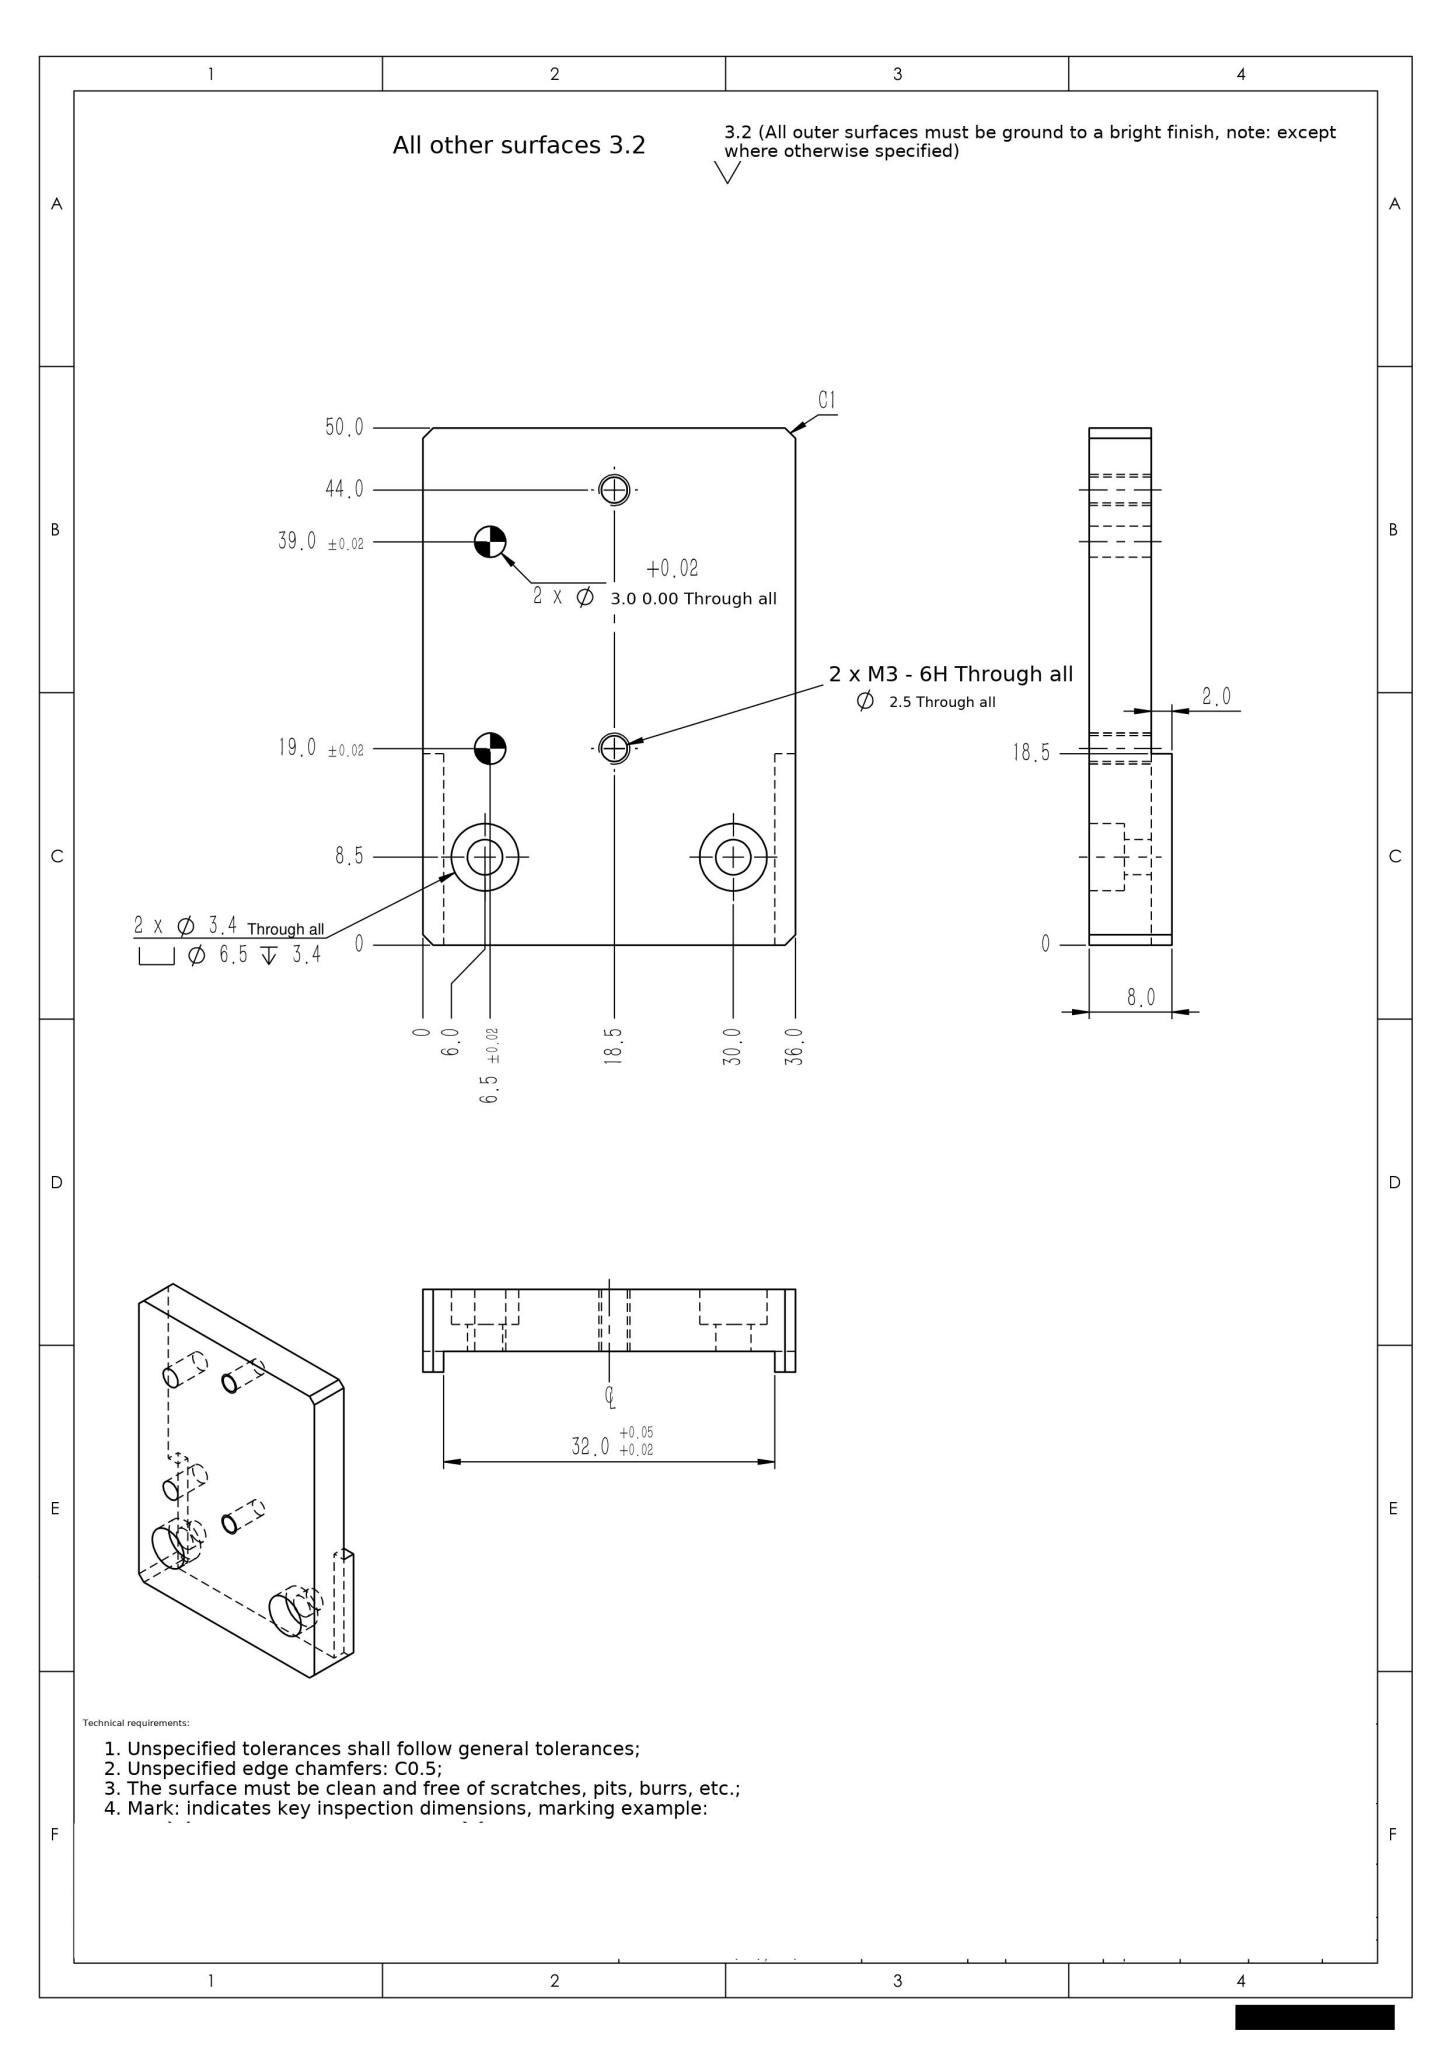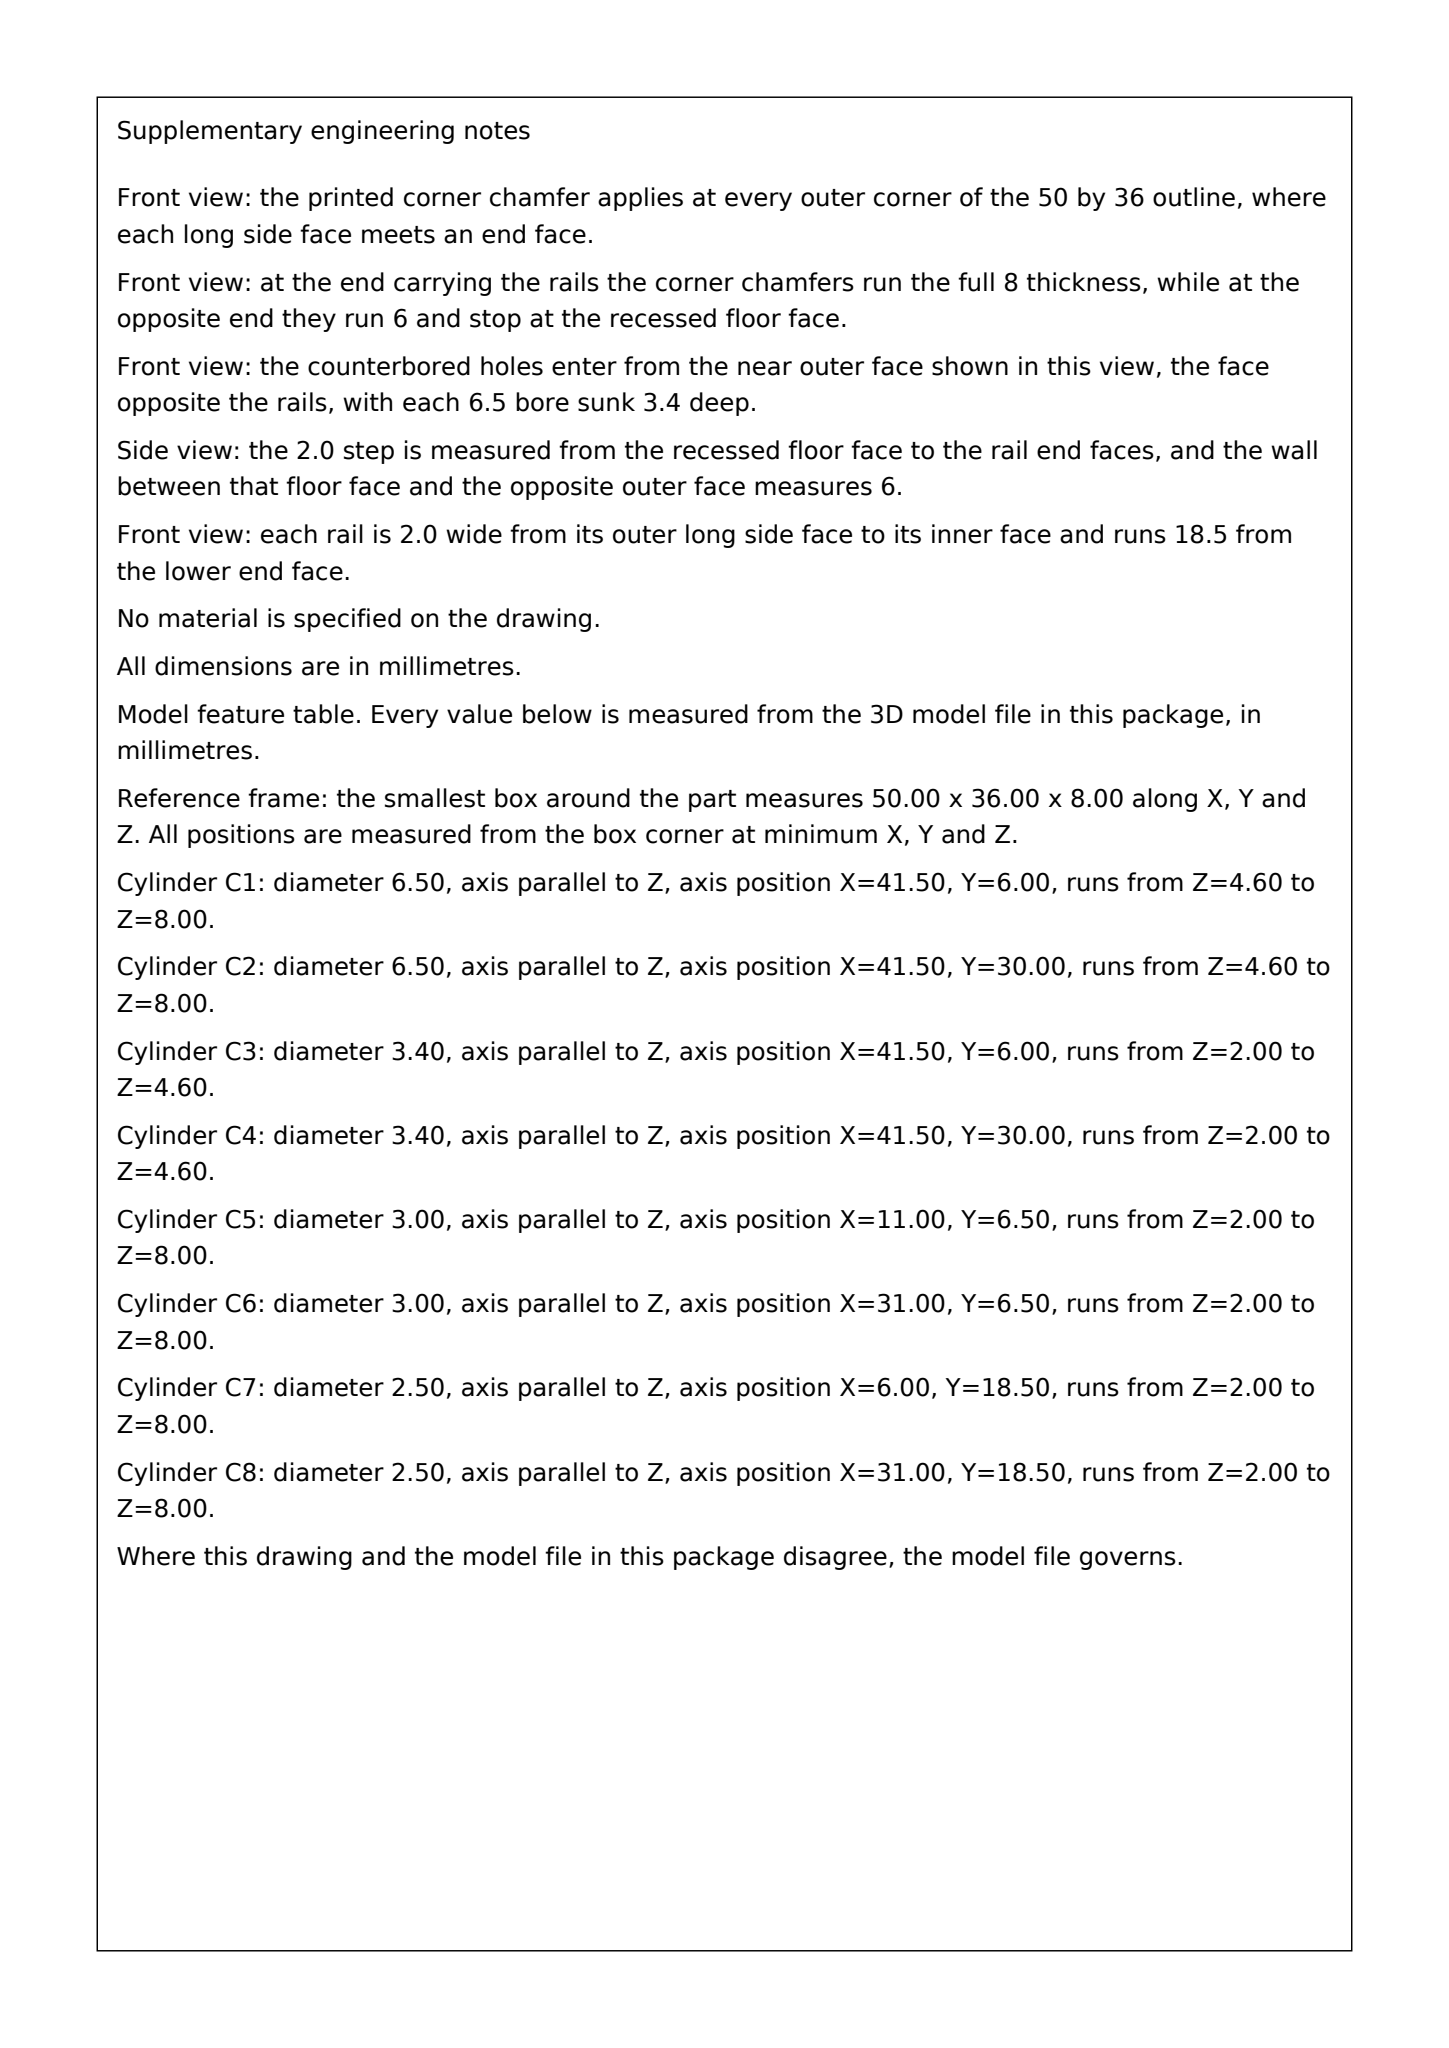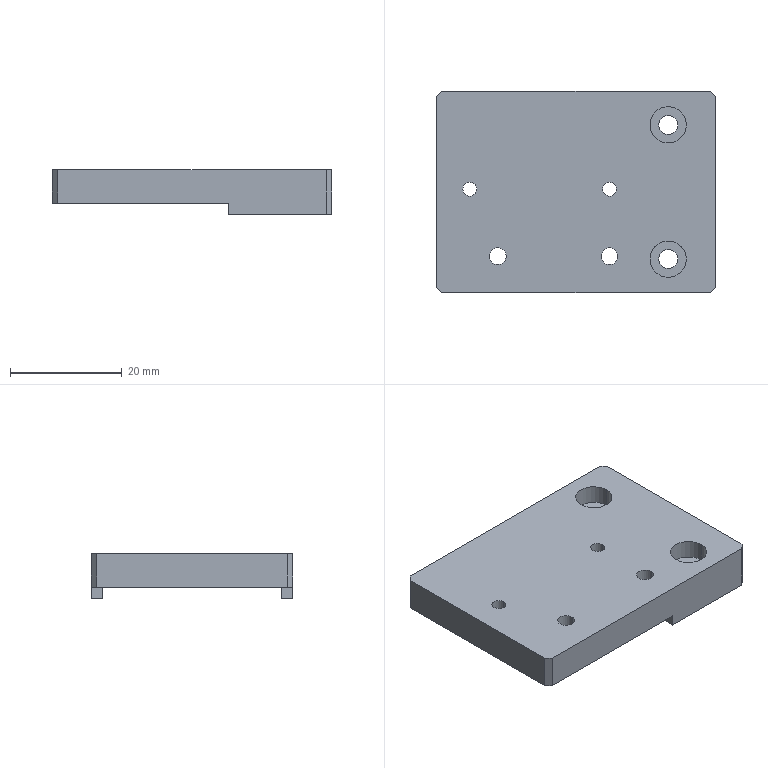Part | SolidWorks | mm | 1 solid | 34 faces | box 50 x 36 x 8 mm | volume 10517 mm3 | plane 18 | cylinder 16 | commonest cylinder face diameters 3 x4 2.5 x4 6.5 x4 3.4 x4
Drawing notes:
2 X Ø3.0 +0.02/0 THRU ALL | from the solid: Two ø3.0 z-axis cylinders at (11.0,6.5) and (31.0,6.5), length 6.0 thru plate
build123d program:
from build123d import *

# Parameters (mm, degrees)
SKETCH1_W                                       = 50
SKETCH1_H                                       = 36
BOSS_EXTRUDE1_DEPTH                             = 8
M3_HEX_SOCKET_HEAD_CAP_SCREW_CBORE1_D           = 3.4
M3_HEX_SOCKET_HEAD_CAP_SCREW_CBORE1_CBORE_D     = 6.5
M3_HEX_SOCKET_HEAD_CAP_SCREW_CBORE1_CBORE_DEPTH = 3.4
M3_TAPPED_HOLE1_D                               = 2.5
SIZE_MM_DOWEL_PIN_HOLE2_D                       = 3
LPATTERN1_COUNT                                 = 2
LPATTERN1_PITCH                                 = 20
SKETCH15_W                                      = 2
SKETCH15_H                                      = 32
CUT_EXTRUDE1_DEPTH                              = 54.74
CHAMFER1_SIZE                                   = 1
SKETCH16_W                                      = 31.5
SKETCH16_H                                      = 36
CUT_EXTRUDE2_DEPTH                              = 2


with BuildPart() as part:
    # Sketch1 → Boss-Extrude1 (new body)
    with BuildSketch(Plane.XY):
        Rectangle(SKETCH1_W, SKETCH1_H)
    extrude(amount=BOSS_EXTRUDE1_DEPTH)

    # M3 Hex Socket Head Cap Screw CBORE1 (through all)
    with Locations(Plane.XY.offset(8)):
        with Locations((16.5, -12), (16.5, 12)):
            CounterBoreHole(M3_HEX_SOCKET_HEAD_CAP_SCREW_CBORE1_D / 2, M3_HEX_SOCKET_HEAD_CAP_SCREW_CBORE1_CBORE_D / 2, M3_HEX_SOCKET_HEAD_CAP_SCREW_CBORE1_CBORE_DEPTH)

    # M3 Tapped Hole1 (through all)
    with Locations(Plane.XY.offset(8)):
        with Locations((-19, 0.5), (6, 0.5)):
            Hole(M3_TAPPED_HOLE1_D / 2)

    # Size mm Dowel Pin Hole2 (through all)
    with Locations(Plane.XY.offset(8)):
        with Locations((6, -11.5)):
            size_mm_dowel_pin_hole2 = Hole(SIZE_MM_DOWEL_PIN_HOLE2_D / 2)

    # LPattern1: Size mm Dowel Pin Hole2 ×2
    with Locations(*[(-i * LPATTERN1_PITCH, 0, 0) for i in range(1, LPATTERN1_COUNT)]):
        add(size_mm_dowel_pin_hole2, mode=Mode.SUBTRACT)

    # Sketch15 → Cut-Extrude1 (cut, through all)
    with BuildSketch(Plane(origin=(25, 0, 0), x_dir=(0, 0, -1), z_dir=(1, 0, 0))):
        with Locations((-1, 0)):
            Rectangle(SKETCH15_W, SKETCH15_H)
    extrude(amount=-CUT_EXTRUDE1_DEPTH, mode=Mode.SUBTRACT)

    # Chamfer1
    chamfer1_edges = [part.edges().sort_by_distance(p)[0] for p in [
        (25, -18, 4),
        (-25, -18, 4),
        (-25, 18, 4),
        (25, 18, 4),
    ]]
    chamfer(chamfer1_edges, length=CHAMFER1_SIZE)

    # Sketch16 → Cut-Extrude2 (cut)
    with BuildSketch(Plane(origin=(0, 0, 0), x_dir=(-1, 0, 0), z_dir=(0, 0, -1))):
        with Locations((9.25, 0)):
            Rectangle(SKETCH16_W, SKETCH16_H)
    extrude(amount=-CUT_EXTRUDE2_DEPTH, mode=Mode.SUBTRACT)


solid = part.part